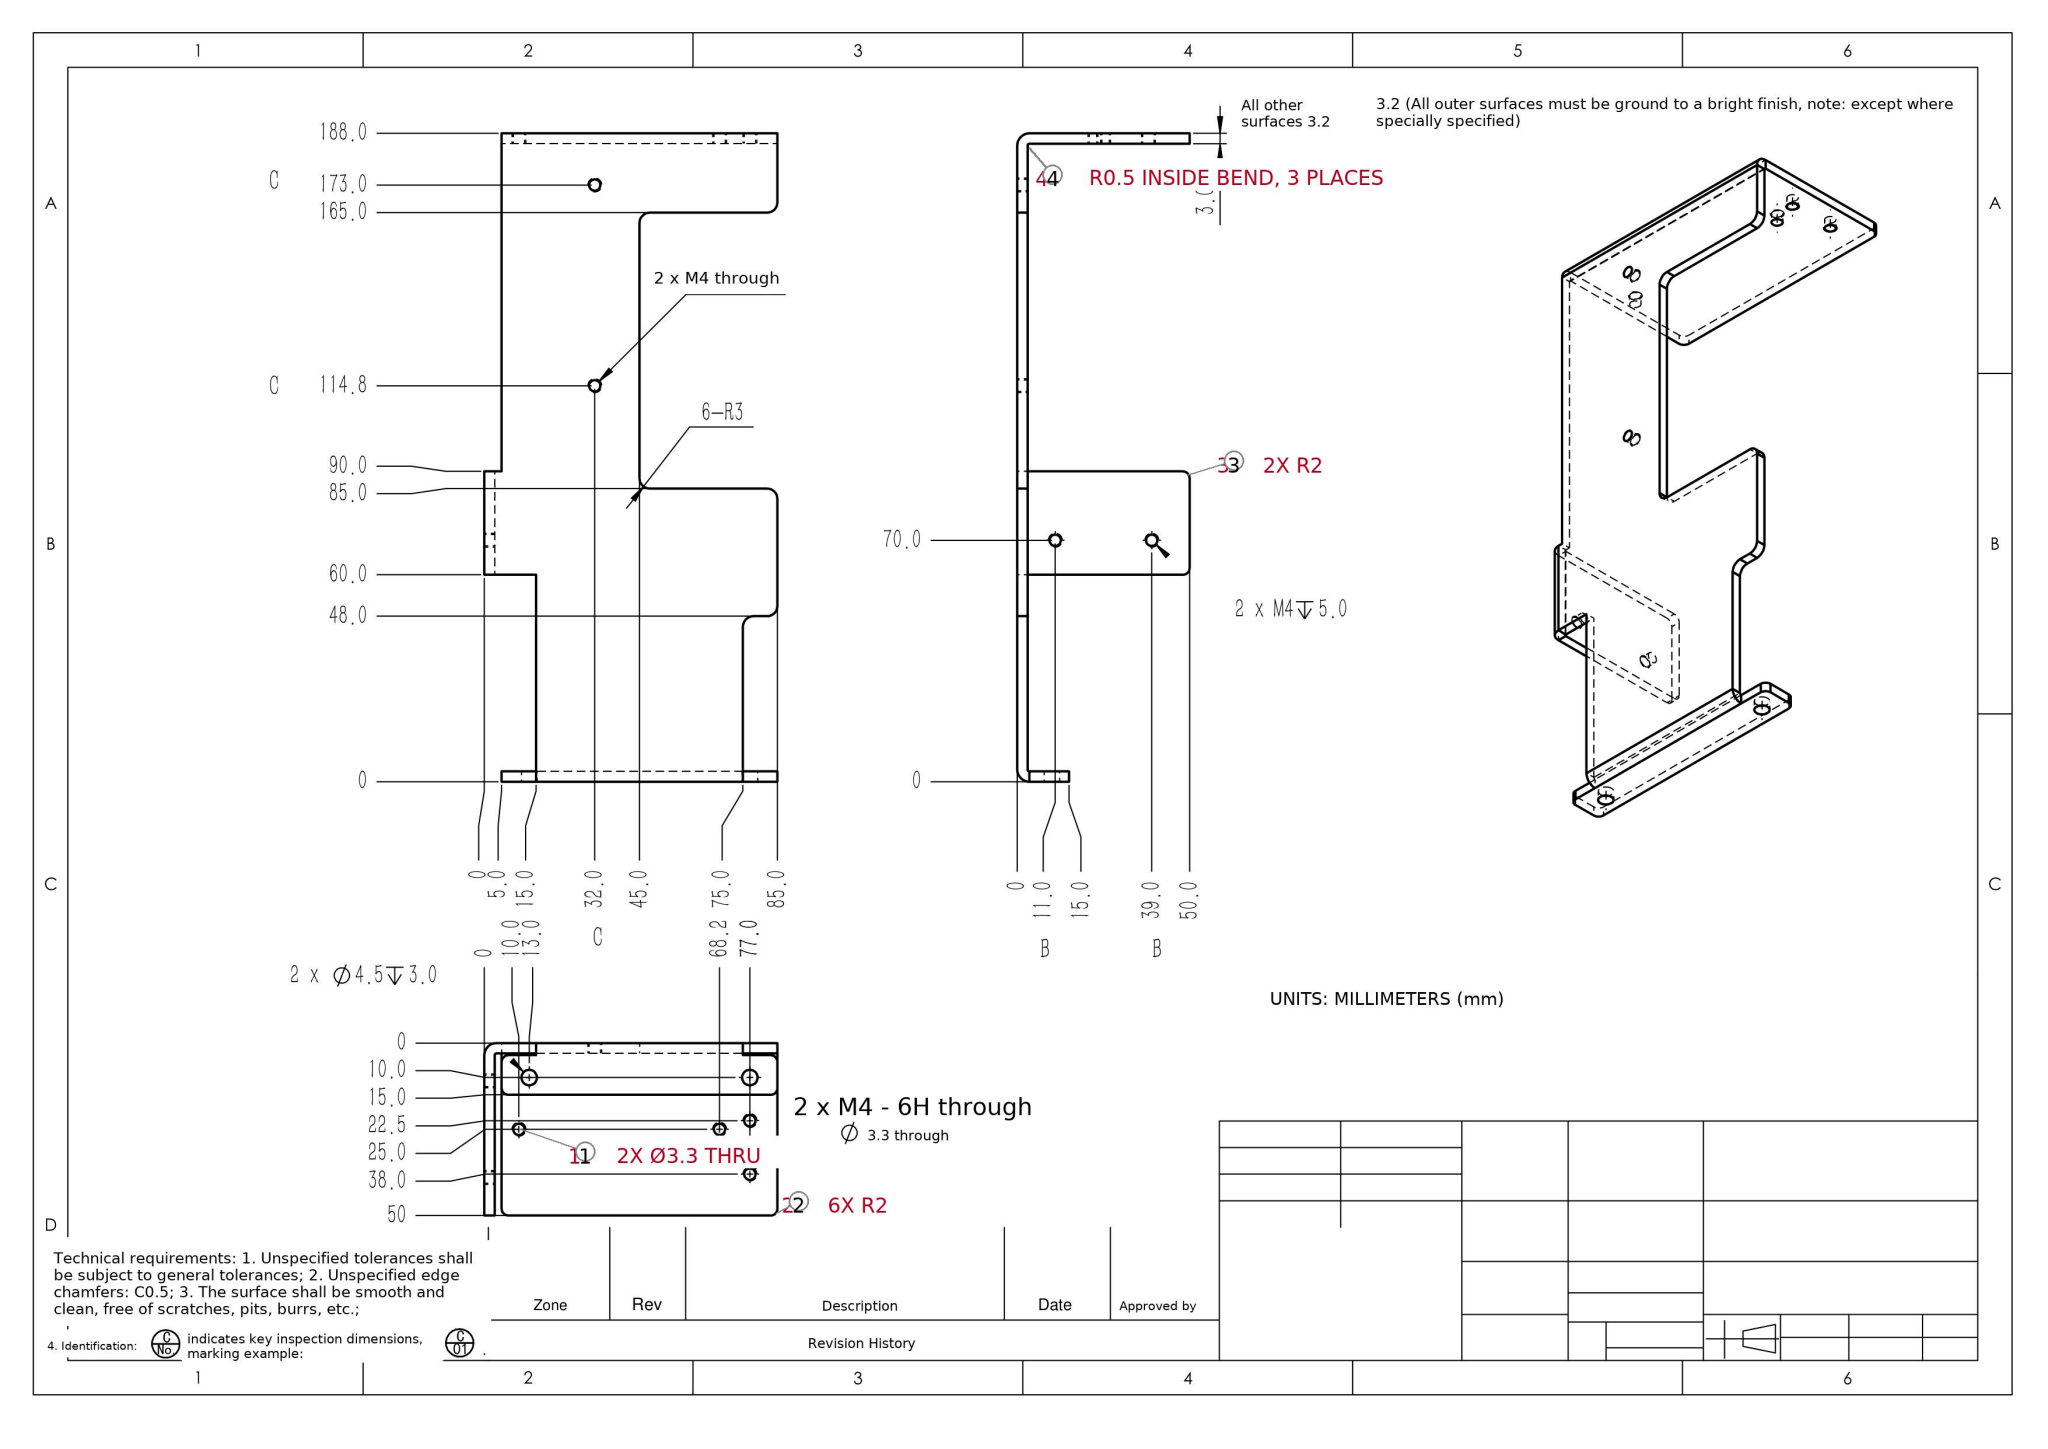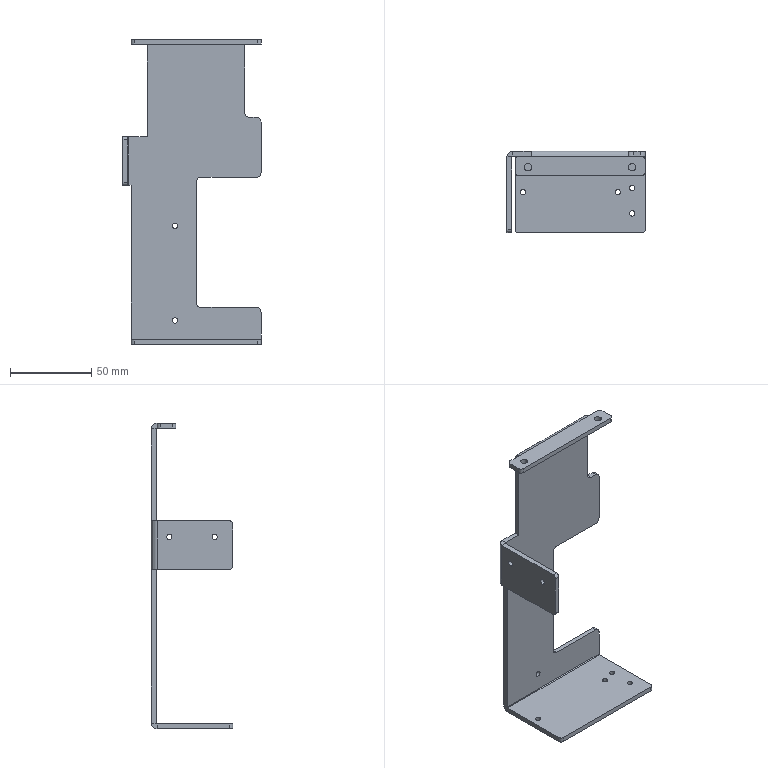Part | SolidWorks | mm | 1 solid | 76 faces | box 85 x 50 x 188 mm | volume 50331 mm3 | cylinder 40 | plane 36 | commonest cylinder face diameters 3.3 x16 4 x8 6 x6 4.5 x4 7 x3 1 x3